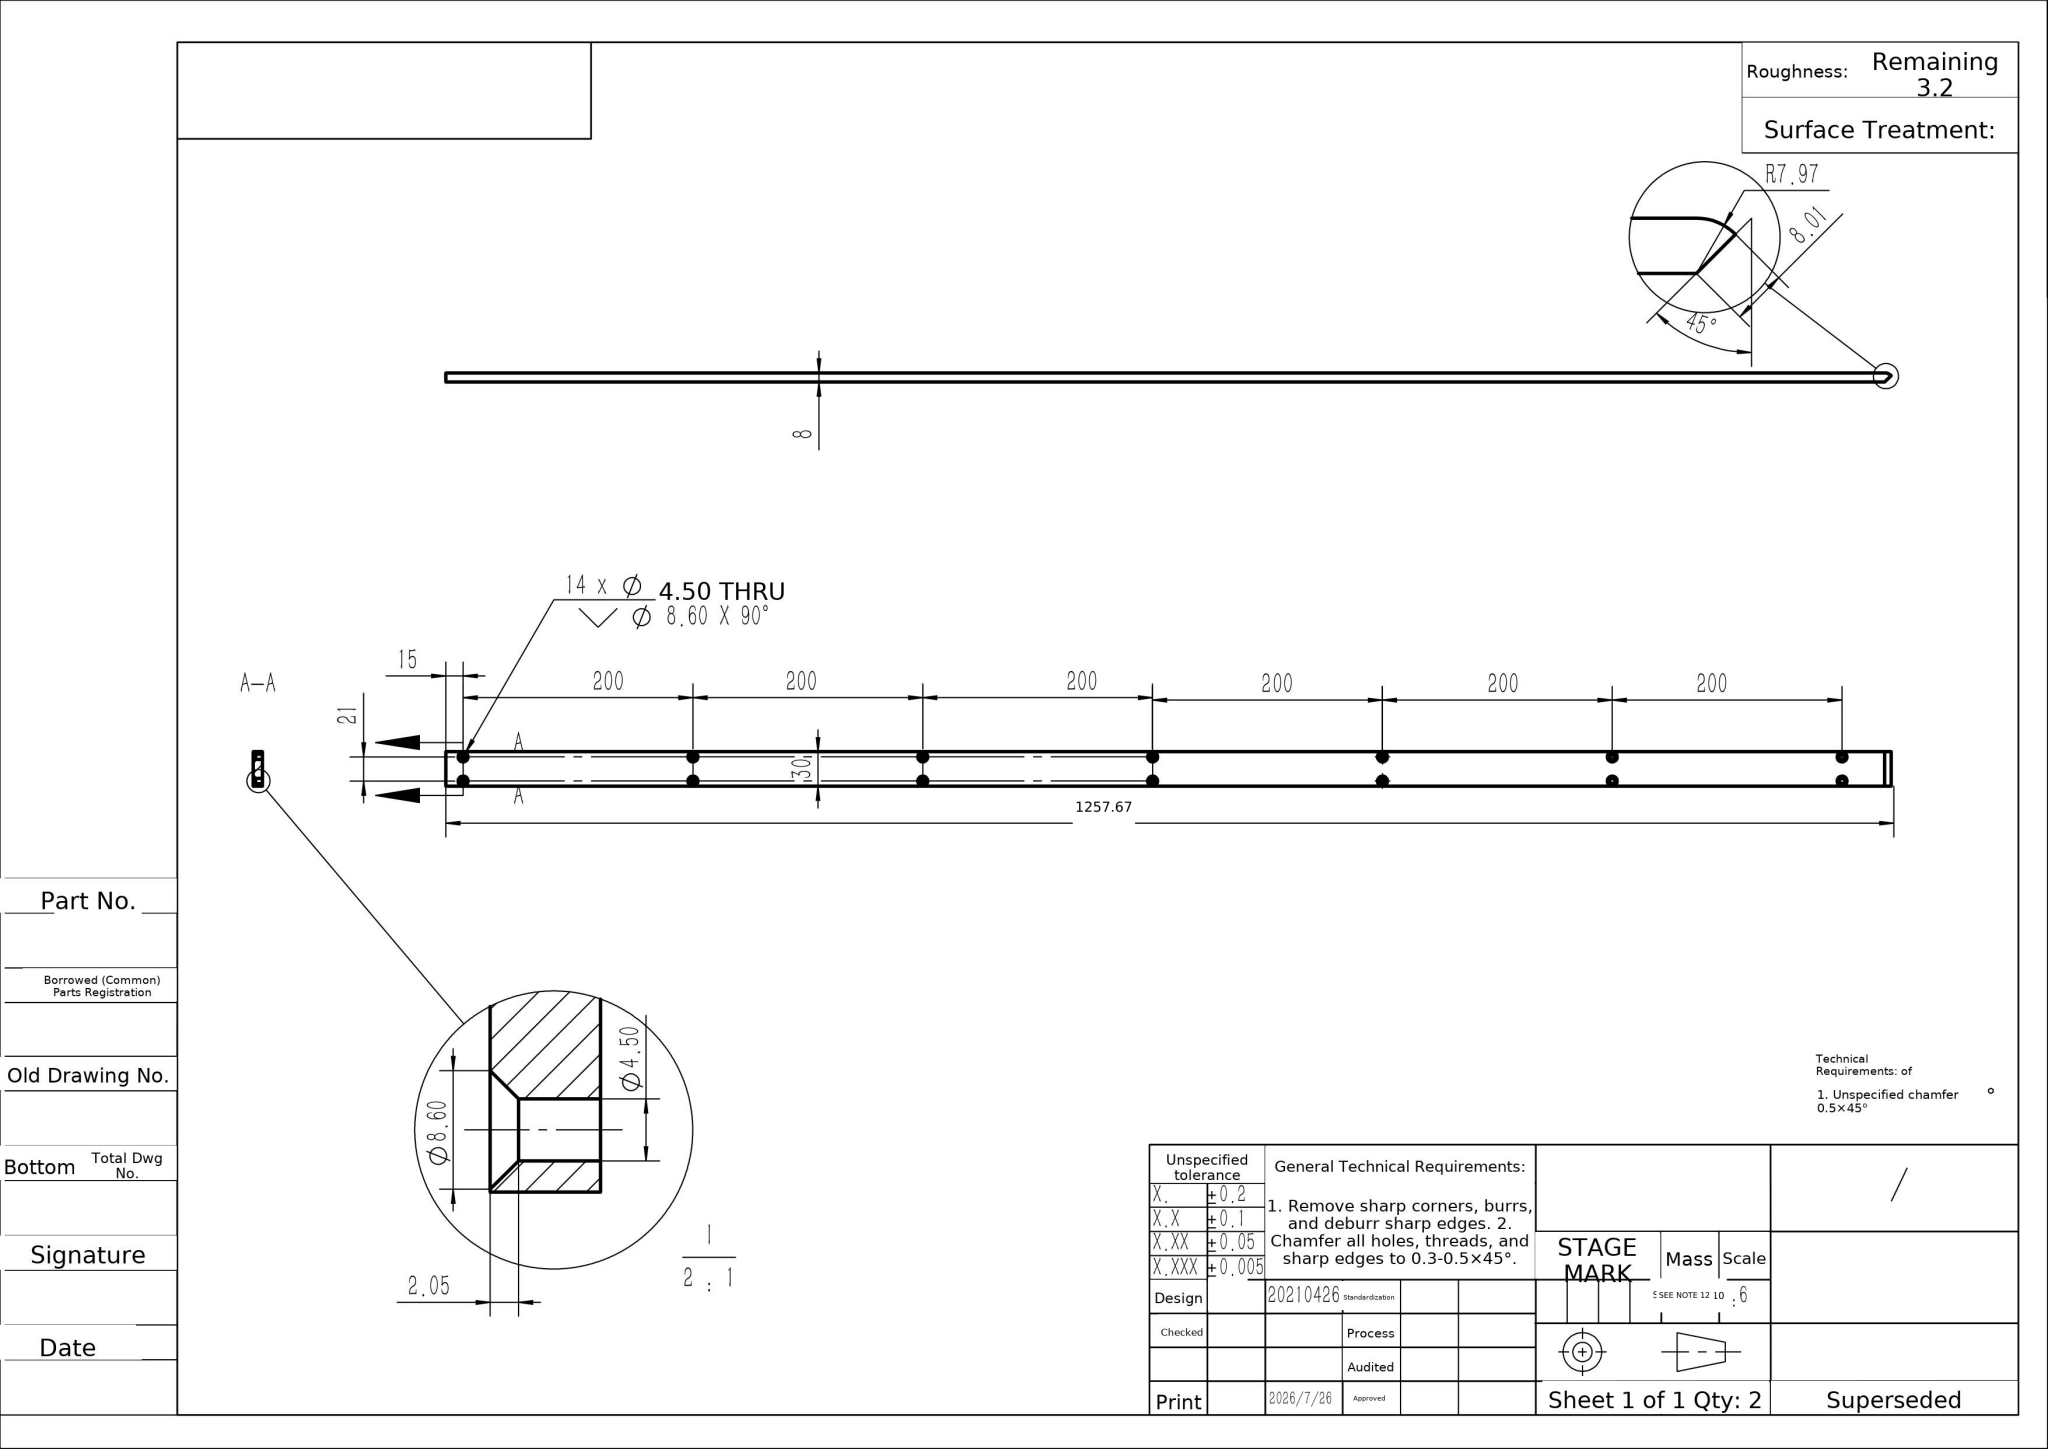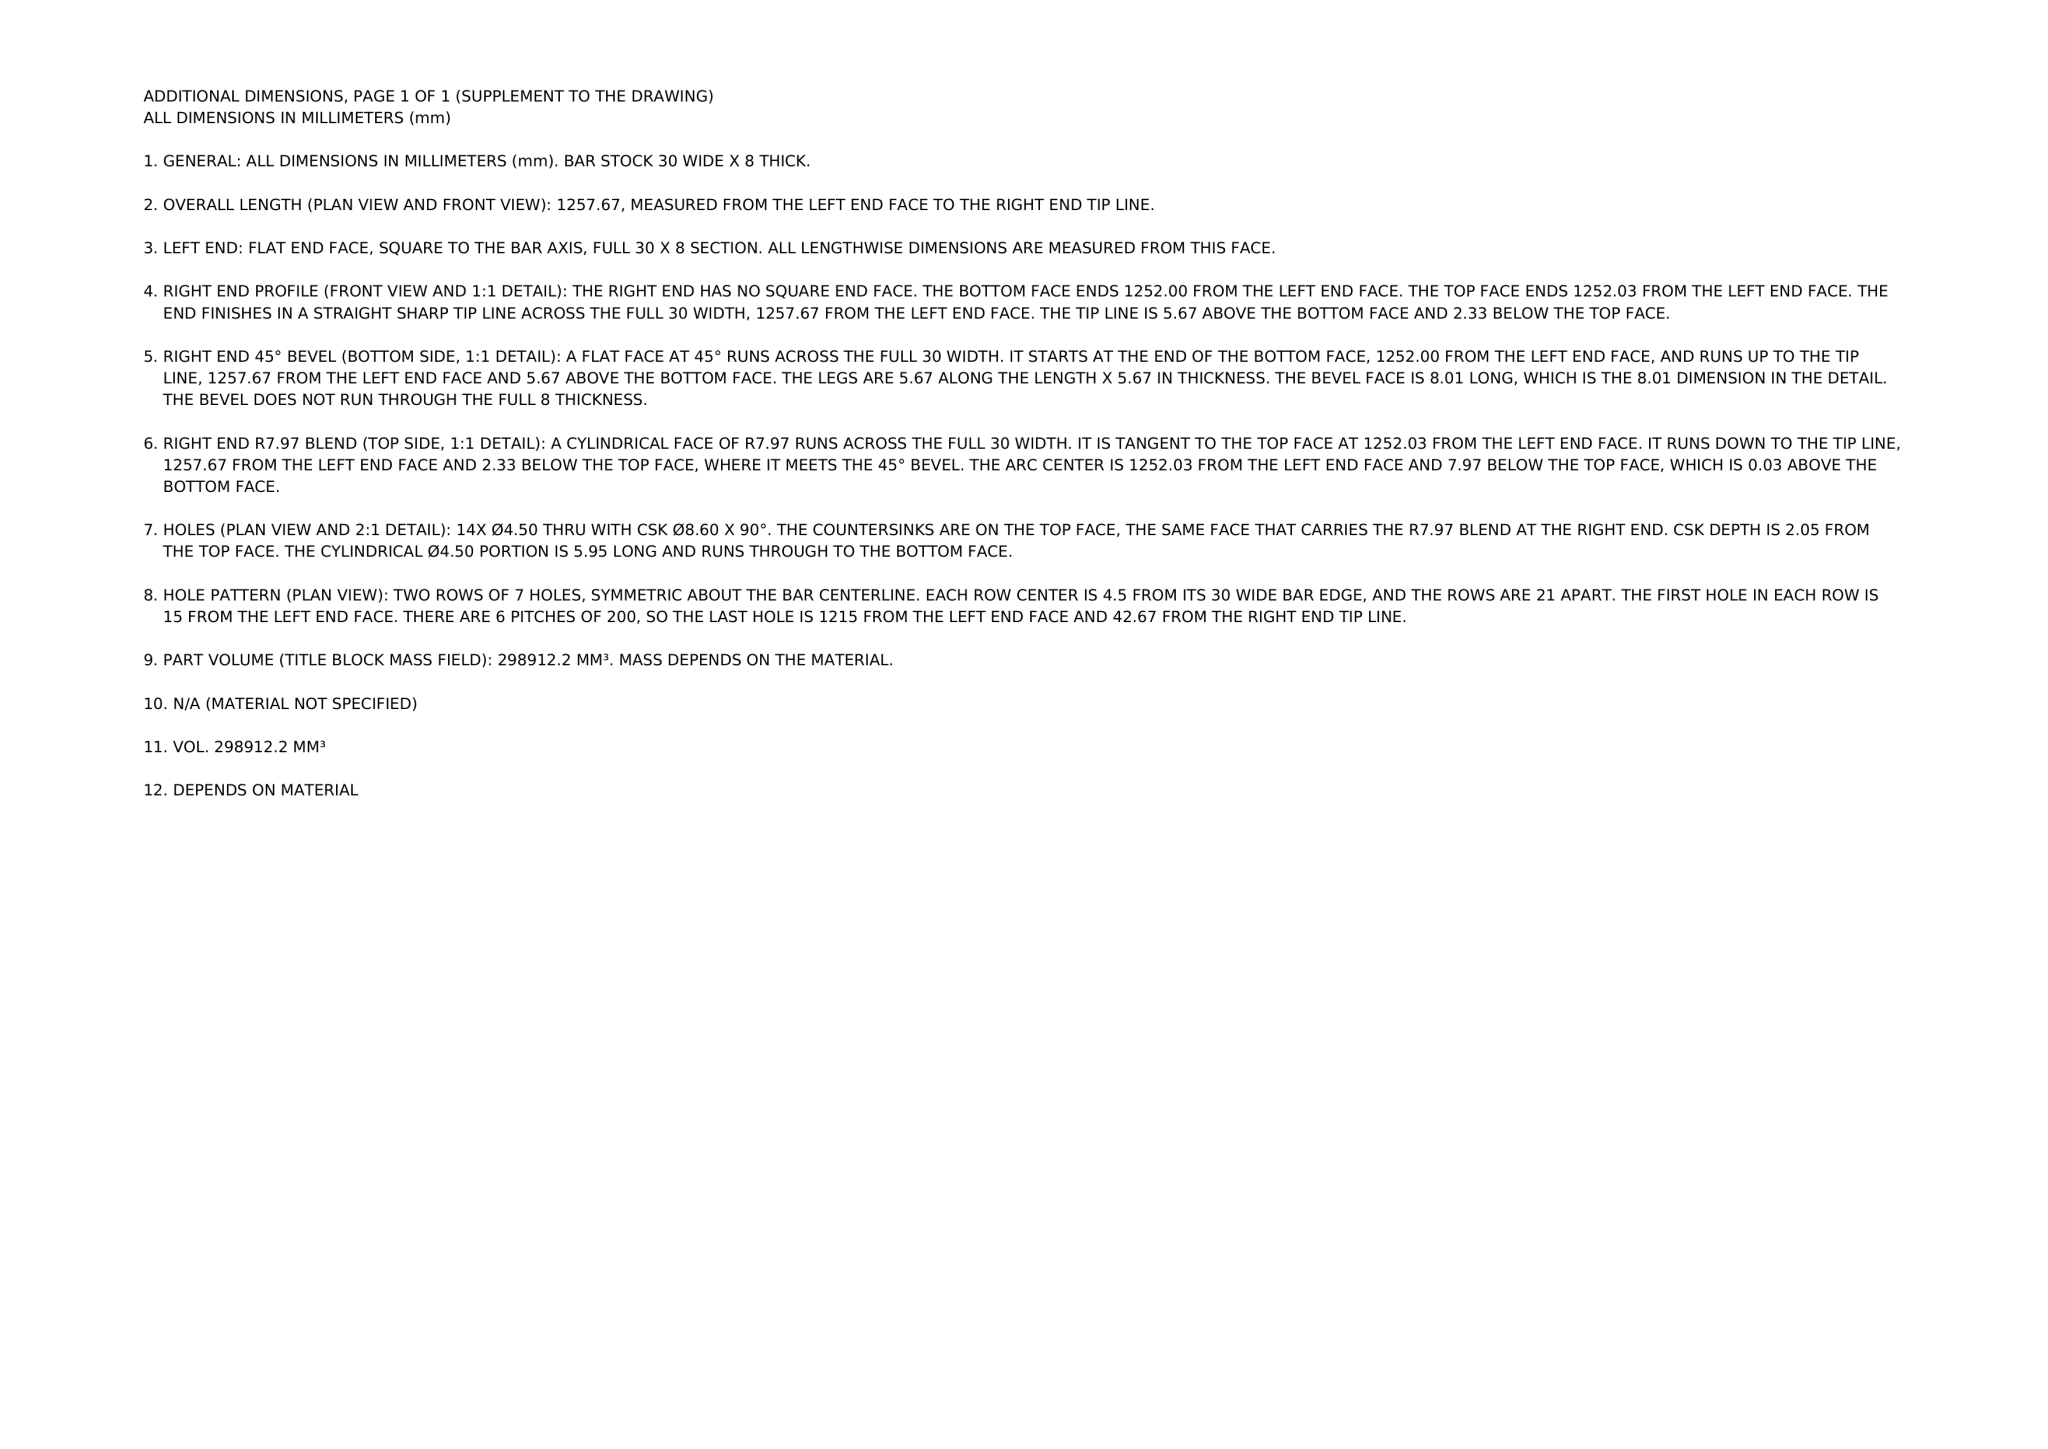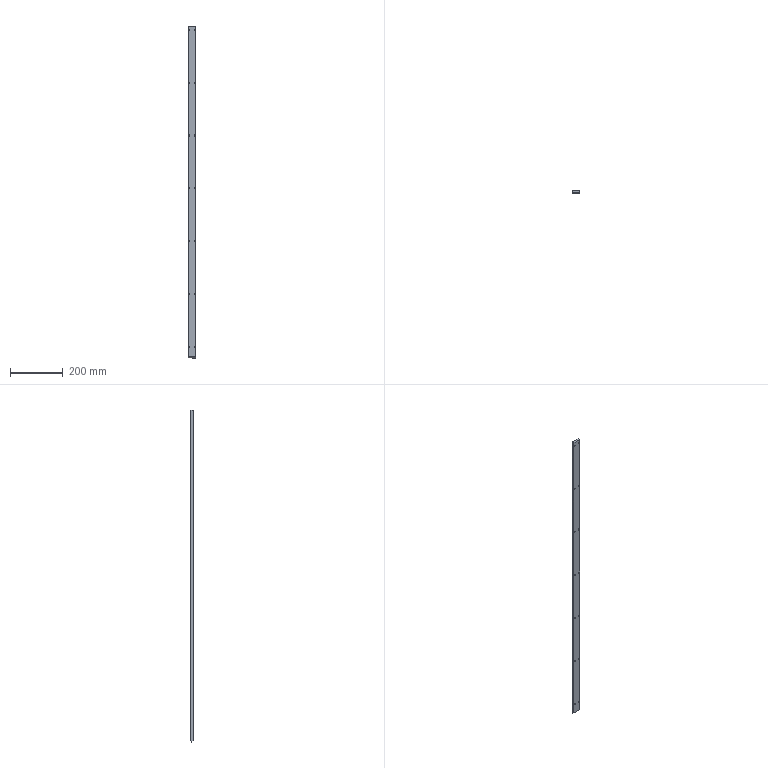Part | NX | mm | 1 solid | 63 faces | box 30 x 8 x 1257.67 mm | volume 298912 mm3 | cylinder 29 | cone 28 | plane 6 | commonest cylinder face diameters 4.5 x28 15.934 x1